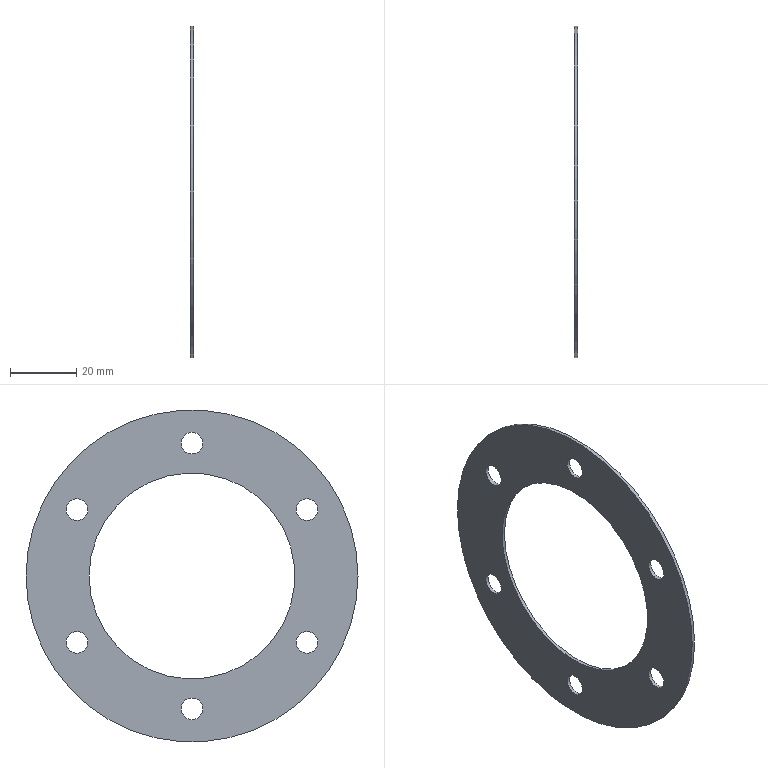Component | NX | DADIANPIAN | 1 solid | 10 faces | box 1 x 100 x 100 mm | volume 4636 mm3 | cylinder 8 | plane 2 | commonest cylinder face diameters 6.5 x6 100 x1 62 x1
STEP:
#1=CARTESIAN_POINT('',(0.,0.,0.));
#2=DIRECTION('',(0.,0.,1.));
#3=DIRECTION('',(1.,0.,0.));
#4=AXIS2_PLACEMENT_3D('',#1,#2,#3);
#5=CARTESIAN_POINT('',(111.,250.,-88.));
#6=VERTEX_POINT('',#5);
#7=CARTESIAN_POINT('',(111.,200.,-88.));
#8=DIRECTION('',(1.,0.,0.));
#9=DIRECTION('',(0.,1.,0.));
#10=AXIS2_PLACEMENT_3D('',#7,#8,#9);
#11=CIRCLE('',#10,50.);
#12=CARTESIAN_POINT('',(111.,200.,-88.));
#13=DIRECTION('',(-1.,0.,0.));
#14=DIRECTION('',(0.,0.,1.));
#15=AXIS2_PLACEMENT_3D('',#12,#13,#14);
#16=CYLINDRICAL_SURFACE('',#15,50.);
#17=CARTESIAN_POINT('',(7.854,0.));
#18=DIRECTION('',(-1.,0.));
#19=VECTOR('',#18,1.);
#20=LINE('',#17,#19);
#21=(GEOMETRIC_REPRESENTATION_CONTEXT(2)PARAMETRIC_REPRESENTATION_CONTEXT()REPRESENTATION_CONTEXT('',''));
#22=DEFINITIONAL_REPRESENTATION('',(#20),#21);
#23=PCURVE('',#16,#22);
#24=CARTESIAN_POINT('',(111.,200.,-88.));
#25=DIRECTION('',(1.,0.,0.));
#26=DIRECTION('',(0.,0.,-1.));
#27=AXIS2_PLACEMENT_3D('',#24,#25,#26);
#28=PLANE('',#27);
#29=CARTESIAN_POINT('',(0.,0.));
#30=DIRECTION('',(0.,1.));
#31=AXIS2_PLACEMENT_2D('',#29,#30);
#32=CIRCLE('',#31,50.);
#33=(GEOMETRIC_REPRESENTATION_CONTEXT(2)PARAMETRIC_REPRESENTATION_CONTEXT()REPRESENTATION_CONTEXT('',''));
#34=DEFINITIONAL_REPRESENTATION('',(#32),#33);
#35=PCURVE('',#28,#34);
#36=SURFACE_CURVE('',#11,(#23,#35),.PCURVE_S1.);
#37=EDGE_CURVE('',#6,#6,#36,.T.);
#38=ORIENTED_EDGE('',*,*,#37,.F.);
#39=CARTESIAN_POINT('',(110.,250.,-88.));
#40=VERTEX_POINT('',#39);
#41=CARTESIAN_POINT('',(111.,250.,-88.));
#42=CARTESIAN_POINT('',(110.,250.,-88.));
#43=B_SPLINE_CURVE_WITH_KNOTS('',1,(#41,#42),.UNSPECIFIED.,.F.,.F.,(2,2),(0.,1.),.PIECEWISE_BEZIER_KNOTS.);
#44=CARTESIAN_POINT('',(7.854,0.));
#45=DIRECTION('',(0.,1.));
#46=VECTOR('',#45,1.);
#47=LINE('',#44,#46);
#48=(GEOMETRIC_REPRESENTATION_CONTEXT(2)PARAMETRIC_REPRESENTATION_CONTEXT()REPRESENTATION_CONTEXT('',''));
#49=DEFINITIONAL_REPRESENTATION('',(#47),#48);
#50=PCURVE('',#16,#49);
#51=CARTESIAN_POINT('',(1.571,0.));
#52=DIRECTION('',(0.,1.));
#53=VECTOR('',#52,1.);
#54=LINE('',#51,#53);
#55=(GEOMETRIC_REPRESENTATION_CONTEXT(2)PARAMETRIC_REPRESENTATION_CONTEXT()REPRESENTATION_CONTEXT('',''));
#56=DEFINITIONAL_REPRESENTATION('',(#54),#55);
#57=PCURVE('',#16,#56);
#58=SEAM_CURVE('',#43,(#50,#57),.PCURVE_S1.);
#59=EDGE_CURVE('',#6,#40,#58,.T.);
#60=ORIENTED_EDGE('',*,*,#59,.T.);
#61=CARTESIAN_POINT('',(110.,200.,-88.));
#62=DIRECTION('',(1.,0.,0.));
#63=DIRECTION('',(0.,1.,0.));
#64=AXIS2_PLACEMENT_3D('',#61,#62,#63);
#65=CIRCLE('',#64,50.);
#66=CARTESIAN_POINT('',(7.854,1.));
#67=DIRECTION('',(-1.,0.));
#68=VECTOR('',#67,1.);
#69=LINE('',#66,#68);
#70=(GEOMETRIC_REPRESENTATION_CONTEXT(2)PARAMETRIC_REPRESENTATION_CONTEXT()REPRESENTATION_CONTEXT('',''));
#71=DEFINITIONAL_REPRESENTATION('',(#69),#70);
#72=PCURVE('',#16,#71);
#73=CARTESIAN_POINT('',(110.,200.,-88.));
#74=DIRECTION('',(1.,0.,0.));
#75=DIRECTION('',(0.,0.,-1.));
#76=AXIS2_PLACEMENT_3D('',#73,#74,#75);
#77=PLANE('',#76);
#78=CARTESIAN_POINT('',(0.,0.));
#79=DIRECTION('',(0.,1.));
#80=AXIS2_PLACEMENT_2D('',#78,#79);
#81=CIRCLE('',#80,50.);
#82=(GEOMETRIC_REPRESENTATION_CONTEXT(2)PARAMETRIC_REPRESENTATION_CONTEXT()REPRESENTATION_CONTEXT('',''));
#83=DEFINITIONAL_REPRESENTATION('',(#81),#82);
#84=PCURVE('',#77,#83);
#85=SURFACE_CURVE('',#65,(#72,#84),.PCURVE_S1.);
#86=EDGE_CURVE('',#40,#40,#85,.T.);
#87=ORIENTED_EDGE('',*,*,#86,.T.);
#88=ORIENTED_EDGE('',*,*,#59,.F.);
#89=EDGE_LOOP('',(#38,#60,#87,#88));
#90=FACE_BOUND('',#89,.T.);
#91=ADVANCED_FACE('',(#90),#16,.T.);
#92=CARTESIAN_POINT('',(111.,231.,-88.));
#93=VERTEX_POINT('',#92);
#94=CARTESIAN_POINT('',(111.,200.,-88.));
#95=DIRECTION('',(1.,0.,0.));
#96=DIRECTION('',(0.,1.,0.));
#97=AXIS2_PLACEMENT_3D('',#94,#95,#96);
#98=CIRCLE('',#97,31.);
#99=CARTESIAN_POINT('',(111.,200.,-88.));
#100=DIRECTION('',(-1.,0.,0.));
#101=DIRECTION('',(0.,0.,1.));
#102=AXIS2_PLACEMENT_3D('',#99,#100,#101);
#103=CYLINDRICAL_SURFACE('',#102,31.);
#104=CARTESIAN_POINT('',(7.854,0.));
#105=DIRECTION('',(-1.,0.));
#106=VECTOR('',#105,1.);
#107=LINE('',#104,#106);
#108=(GEOMETRIC_REPRESENTATION_CONTEXT(2)PARAMETRIC_REPRESENTATION_CONTEXT()REPRESENTATION_CONTEXT('',''));
#109=DEFINITIONAL_REPRESENTATION('',(#107),#108);
#110=PCURVE('',#103,#109);
#111=CARTESIAN_POINT('',(0.,0.));
#112=DIRECTION('',(0.,1.));
#113=AXIS2_PLACEMENT_2D('',#111,#112);
#114=CIRCLE('',#113,31.);
#115=(GEOMETRIC_REPRESENTATION_CONTEXT(2)PARAMETRIC_REPRESENTATION_CONTEXT()REPRESENTATION_CONTEXT('',''));
#116=DEFINITIONAL_REPRESENTATION('',(#114),#115);
#117=PCURVE('',#28,#116);
#118=SURFACE_CURVE('',#98,(#110,#117),.PCURVE_S1.);
#119=EDGE_CURVE('',#93,#93,#118,.T.);
#120=ORIENTED_EDGE('',*,*,#119,.F.);
#121=CARTESIAN_POINT('',(110.,231.,-88.));
#122=VERTEX_POINT('',#121);
#123=CARTESIAN_POINT('',(111.,231.,-88.));
#124=CARTESIAN_POINT('',(110.,231.,-88.));
#125=B_SPLINE_CURVE_WITH_KNOTS('',1,(#123,#124),.UNSPECIFIED.,.F.,.F.,(2,2),(0.,1.),.PIECEWISE_BEZIER_KNOTS.);
#126=CARTESIAN_POINT('',(7.854,0.));
#127=DIRECTION('',(0.,1.));
#128=VECTOR('',#127,1.);
#129=LINE('',#126,#128);
#130=(GEOMETRIC_REPRESENTATION_CONTEXT(2)PARAMETRIC_REPRESENTATION_CONTEXT()REPRESENTATION_CONTEXT('',''));
#131=DEFINITIONAL_REPRESENTATION('',(#129),#130);
#132=PCURVE('',#103,#131);
#133=CARTESIAN_POINT('',(1.571,0.));
#134=DIRECTION('',(0.,1.));
#135=VECTOR('',#134,1.);
#136=LINE('',#133,#135);
#137=(GEOMETRIC_REPRESENTATION_CONTEXT(2)PARAMETRIC_REPRESENTATION_CONTEXT()REPRESENTATION_CONTEXT('',''));
#138=DEFINITIONAL_REPRESENTATION('',(#136),#137);
#139=PCURVE('',#103,#138);
#140=SEAM_CURVE('',#125,(#132,#139),.PCURVE_S1.);
#141=EDGE_CURVE('',#93,#122,#140,.T.);
#142=ORIENTED_EDGE('',*,*,#141,.T.);
#143=CARTESIAN_POINT('',(110.,200.,-88.));
#144=DIRECTION('',(1.,0.,0.));
#145=DIRECTION('',(0.,1.,0.));
#146=AXIS2_PLACEMENT_3D('',#143,#144,#145);
#147=CIRCLE('',#146,31.);
#148=CARTESIAN_POINT('',(7.854,1.));
#149=DIRECTION('',(-1.,0.));
#150=VECTOR('',#149,1.);
#151=LINE('',#148,#150);
#152=(GEOMETRIC_REPRESENTATION_CONTEXT(2)PARAMETRIC_REPRESENTATION_CONTEXT()REPRESENTATION_CONTEXT('',''));
#153=DEFINITIONAL_REPRESENTATION('',(#151),#152);
#154=PCURVE('',#103,#153);
#155=CARTESIAN_POINT('',(0.,0.));
#156=DIRECTION('',(0.,1.));
#157=AXIS2_PLACEMENT_2D('',#155,#156);
#158=CIRCLE('',#157,31.);
#159=(GEOMETRIC_REPRESENTATION_CONTEXT(2)PARAMETRIC_REPRESENTATION_CONTEXT()REPRESENTATION_CONTEXT('',''));
#160=DEFINITIONAL_REPRESENTATION('',(#158),#159);
#161=PCURVE('',#77,#160);
#162=SURFACE_CURVE('',#147,(#154,#161),.PCURVE_S1.);
#163=EDGE_CURVE('',#122,#122,#162,.T.);
#164=ORIENTED_EDGE('',*,*,#163,.T.);
#165=ORIENTED_EDGE('',*,*,#141,.F.);
#166=EDGE_LOOP('',(#120,#142,#164,#165));
#167=FACE_BOUND('',#166,.F.);
#168=ADVANCED_FACE('',(#167),#103,.F.);
#169=CARTESIAN_POINT('',(111.,234.641,-64.75));
#170=VERTEX_POINT('',#169);
#171=CARTESIAN_POINT('',(111.,234.641,-68.));
#172=DIRECTION('',(-1.,0.,0.));
#173=DIRECTION('',(0.,0.,1.));
#174=AXIS2_PLACEMENT_3D('',#171,#172,#173);
#175=CIRCLE('',#174,3.25);
#176=CARTESIAN_POINT('',(-23.25,34.641));
#177=CARTESIAN_POINT('',(-23.25,40.27));
#178=CARTESIAN_POINT('',(-18.375,37.456));
#179=CARTESIAN_POINT('',(-13.5,34.641));
#180=CARTESIAN_POINT('',(-18.375,31.826));
#181=CARTESIAN_POINT('',(-23.25,29.012));
#182=CARTESIAN_POINT('',(-23.25,34.641));
#183=(BOUNDED_CURVE()B_SPLINE_CURVE(2,(#176,#177,#178,#179,#180,#181,#182),.UNSPECIFIED.,.T.,.F.)B_SPLINE_CURVE_WITH_KNOTS((1,2,2,2,2,1),(-2.094,0.,2.094,4.189,6.283,8.378),.UNSPECIFIED.)CURVE()GEOMETRIC_REPRESENTATION_ITEM()RATIONAL_B_SPLINE_CURVE((1.,0.5,1.,0.5,1.,0.5,1.))REPRESENTATION_ITEM(''));
#184=(GEOMETRIC_REPRESENTATION_CONTEXT(2)PARAMETRIC_REPRESENTATION_CONTEXT()REPRESENTATION_CONTEXT('',''));
#185=DEFINITIONAL_REPRESENTATION('',(#183),#184);
#186=PCURVE('',#28,#185);
#187=CARTESIAN_POINT('',(111.,234.641,-68.));
#188=DIRECTION('',(-1.,0.,0.));
#189=DIRECTION('',(0.,0.,1.));
#190=AXIS2_PLACEMENT_3D('',#187,#188,#189);
#191=CYLINDRICAL_SURFACE('',#190,3.25);
#192=CARTESIAN_POINT('',(0.,0.));
#193=DIRECTION('',(1.,0.));
#194=VECTOR('',#193,1.);
#195=LINE('',#192,#194);
#196=(GEOMETRIC_REPRESENTATION_CONTEXT(2)PARAMETRIC_REPRESENTATION_CONTEXT()REPRESENTATION_CONTEXT('',''));
#197=DEFINITIONAL_REPRESENTATION('',(#195),#196);
#198=PCURVE('',#191,#197);
#199=SURFACE_CURVE('',#175,(#186,#198),.PCURVE_S1.);
#200=EDGE_CURVE('',#170,#170,#199,.T.);
#201=ORIENTED_EDGE('',*,*,#200,.T.);
#202=EDGE_LOOP('',(#201));
#203=FACE_BOUND('',#202,.T.);
#204=CARTESIAN_POINT('',(111.,234.641,-104.75));
#205=VERTEX_POINT('',#204);
#206=CARTESIAN_POINT('',(111.,234.641,-108.));
#207=DIRECTION('',(-1.,0.,0.));
#208=DIRECTION('',(0.,0.,1.));
#209=AXIS2_PLACEMENT_3D('',#206,#207,#208);
#210=CIRCLE('',#209,3.25);
#211=CARTESIAN_POINT('',(16.75,34.641));
#212=CARTESIAN_POINT('',(16.75,40.27));
#213=CARTESIAN_POINT('',(21.625,37.456));
#214=CARTESIAN_POINT('',(26.5,34.641));
#215=CARTESIAN_POINT('',(21.625,31.826));
#216=CARTESIAN_POINT('',(16.75,29.012));
#217=CARTESIAN_POINT('',(16.75,34.641));
#218=(BOUNDED_CURVE()B_SPLINE_CURVE(2,(#211,#212,#213,#214,#215,#216,#217),.UNSPECIFIED.,.T.,.F.)B_SPLINE_CURVE_WITH_KNOTS((1,2,2,2,2,1),(-2.094,0.,2.094,4.189,6.283,8.378),.UNSPECIFIED.)CURVE()GEOMETRIC_REPRESENTATION_ITEM()RATIONAL_B_SPLINE_CURVE((1.,0.5,1.,0.5,1.,0.5,1.))REPRESENTATION_ITEM(''));
#219=(GEOMETRIC_REPRESENTATION_CONTEXT(2)PARAMETRIC_REPRESENTATION_CONTEXT()REPRESENTATION_CONTEXT('',''));
#220=DEFINITIONAL_REPRESENTATION('',(#218),#219);
#221=PCURVE('',#28,#220);
#222=CARTESIAN_POINT('',(111.,234.641,-108.));
#223=DIRECTION('',(-1.,0.,0.));
#224=DIRECTION('',(0.,0.,1.));
#225=AXIS2_PLACEMENT_3D('',#222,#223,#224);
#226=CYLINDRICAL_SURFACE('',#225,3.25);
#227=CARTESIAN_POINT('',(0.,0.));
#228=DIRECTION('',(1.,0.));
#229=VECTOR('',#228,1.);
#230=LINE('',#227,#229);
#231=(GEOMETRIC_REPRESENTATION_CONTEXT(2)PARAMETRIC_REPRESENTATION_CONTEXT()REPRESENTATION_CONTEXT('',''));
#232=DEFINITIONAL_REPRESENTATION('',(#230),#231);
#233=PCURVE('',#226,#232);
#234=SURFACE_CURVE('',#210,(#221,#233),.PCURVE_S1.);
#235=EDGE_CURVE('',#205,#205,#234,.T.);
#236=ORIENTED_EDGE('',*,*,#235,.T.);
#237=EDGE_LOOP('',(#236));
#238=FACE_BOUND('',#237,.T.);
#239=CARTESIAN_POINT('',(111.,200.,-44.75));
#240=VERTEX_POINT('',#239);
#241=CARTESIAN_POINT('',(111.,200.,-48.));
#242=DIRECTION('',(-1.,0.,0.));
#243=DIRECTION('',(0.,0.,1.));
#244=AXIS2_PLACEMENT_3D('',#241,#242,#243);
#245=CIRCLE('',#244,3.25);
#246=CARTESIAN_POINT('',(-43.25,0.));
#247=CARTESIAN_POINT('',(-43.25,5.629));
#248=CARTESIAN_POINT('',(-38.375,2.815));
#249=CARTESIAN_POINT('',(-33.5,0.));
#250=CARTESIAN_POINT('',(-38.375,-2.815));
#251=CARTESIAN_POINT('',(-43.25,-5.629));
#252=CARTESIAN_POINT('',(-43.25,0.));
#253=(BOUNDED_CURVE()B_SPLINE_CURVE(2,(#246,#247,#248,#249,#250,#251,#252),.UNSPECIFIED.,.T.,.F.)B_SPLINE_CURVE_WITH_KNOTS((1,2,2,2,2,1),(-2.094,0.,2.094,4.189,6.283,8.378),.UNSPECIFIED.)CURVE()GEOMETRIC_REPRESENTATION_ITEM()RATIONAL_B_SPLINE_CURVE((1.,0.5,1.,0.5,1.,0.5,1.))REPRESENTATION_ITEM(''));
#254=(GEOMETRIC_REPRESENTATION_CONTEXT(2)PARAMETRIC_REPRESENTATION_CONTEXT()REPRESENTATION_CONTEXT('',''));
#255=DEFINITIONAL_REPRESENTATION('',(#253),#254);
#256=PCURVE('',#28,#255);
#257=CARTESIAN_POINT('',(111.,200.,-48.));
#258=DIRECTION('',(-1.,0.,0.));
#259=DIRECTION('',(0.,0.,1.));
#260=AXIS2_PLACEMENT_3D('',#257,#258,#259);
#261=CYLINDRICAL_SURFACE('',#260,3.25);
#262=CARTESIAN_POINT('',(0.,0.));
#263=DIRECTION('',(1.,0.));
#264=VECTOR('',#263,1.);
#265=LINE('',#262,#264);
#266=(GEOMETRIC_REPRESENTATION_CONTEXT(2)PARAMETRIC_REPRESENTATION_CONTEXT()REPRESENTATION_CONTEXT('',''));
#267=DEFINITIONAL_REPRESENTATION('',(#265),#266);
#268=PCURVE('',#261,#267);
#269=SURFACE_CURVE('',#245,(#256,#268),.PCURVE_S1.);
#270=EDGE_CURVE('',#240,#240,#269,.T.);
#271=ORIENTED_EDGE('',*,*,#270,.T.);
#272=EDGE_LOOP('',(#271));
#273=FACE_BOUND('',#272,.T.);
#274=CARTESIAN_POINT('',(111.,200.,-124.75));
#275=VERTEX_POINT('',#274);
#276=CARTESIAN_POINT('',(111.,200.,-128.));
#277=DIRECTION('',(-1.,0.,0.));
#278=DIRECTION('',(0.,0.,1.));
#279=AXIS2_PLACEMENT_3D('',#276,#277,#278);
#280=CIRCLE('',#279,3.25);
#281=CARTESIAN_POINT('',(36.75,0.));
#282=CARTESIAN_POINT('',(36.75,5.629));
#283=CARTESIAN_POINT('',(41.625,2.815));
#284=CARTESIAN_POINT('',(46.5,0.));
#285=CARTESIAN_POINT('',(41.625,-2.815));
#286=CARTESIAN_POINT('',(36.75,-5.629));
#287=CARTESIAN_POINT('',(36.75,0.));
#288=(BOUNDED_CURVE()B_SPLINE_CURVE(2,(#281,#282,#283,#284,#285,#286,#287),.UNSPECIFIED.,.T.,.F.)B_SPLINE_CURVE_WITH_KNOTS((1,2,2,2,2,1),(-2.094,0.,2.094,4.189,6.283,8.378),.UNSPECIFIED.)CURVE()GEOMETRIC_REPRESENTATION_ITEM()RATIONAL_B_SPLINE_CURVE((1.,0.5,1.,0.5,1.,0.5,1.))REPRESENTATION_ITEM(''));
#289=(GEOMETRIC_REPRESENTATION_CONTEXT(2)PARAMETRIC_REPRESENTATION_CONTEXT()REPRESENTATION_CONTEXT('',''));
#290=DEFINITIONAL_REPRESENTATION('',(#288),#289);
#291=PCURVE('',#28,#290);
#292=CARTESIAN_POINT('',(111.,200.,-128.));
#293=DIRECTION('',(-1.,0.,0.));
#294=DIRECTION('',(0.,0.,1.));
#295=AXIS2_PLACEMENT_3D('',#292,#293,#294);
#296=CYLINDRICAL_SURFACE('',#295,3.25);
#297=CARTESIAN_POINT('',(0.,0.));
#298=DIRECTION('',(1.,0.));
#299=VECTOR('',#298,1.);
#300=LINE('',#297,#299);
#301=(GEOMETRIC_REPRESENTATION_CONTEXT(2)PARAMETRIC_REPRESENTATION_CONTEXT()REPRESENTATION_CONTEXT('',''));
#302=DEFINITIONAL_REPRESENTATION('',(#300),#301);
#303=PCURVE('',#296,#302);
#304=SURFACE_CURVE('',#280,(#291,#303),.PCURVE_S1.);
#305=EDGE_CURVE('',#275,#275,#304,.T.);
#306=ORIENTED_EDGE('',*,*,#305,.T.);
#307=EDGE_LOOP('',(#306));
#308=FACE_BOUND('',#307,.T.);
#309=CARTESIAN_POINT('',(111.,165.359,-64.75));
#310=VERTEX_POINT('',#309);
#311=CARTESIAN_POINT('',(111.,165.359,-68.));
#312=DIRECTION('',(-1.,0.,0.));
#313=DIRECTION('',(0.,0.,1.));
#314=AXIS2_PLACEMENT_3D('',#311,#312,#313);
#315=CIRCLE('',#314,3.25);
#316=CARTESIAN_POINT('',(-23.25,-34.641));
#317=CARTESIAN_POINT('',(-23.25,-29.012));
#318=CARTESIAN_POINT('',(-18.375,-31.826));
#319=CARTESIAN_POINT('',(-13.5,-34.641));
#320=CARTESIAN_POINT('',(-18.375,-37.456));
#321=CARTESIAN_POINT('',(-23.25,-40.27));
#322=CARTESIAN_POINT('',(-23.25,-34.641));
#323=(BOUNDED_CURVE()B_SPLINE_CURVE(2,(#316,#317,#318,#319,#320,#321,#322),.UNSPECIFIED.,.T.,.F.)B_SPLINE_CURVE_WITH_KNOTS((1,2,2,2,2,1),(-2.094,0.,2.094,4.189,6.283,8.378),.UNSPECIFIED.)CURVE()GEOMETRIC_REPRESENTATION_ITEM()RATIONAL_B_SPLINE_CURVE((1.,0.5,1.,0.5,1.,0.5,1.))REPRESENTATION_ITEM(''));
#324=(GEOMETRIC_REPRESENTATION_CONTEXT(2)PARAMETRIC_REPRESENTATION_CONTEXT()REPRESENTATION_CONTEXT('',''));
#325=DEFINITIONAL_REPRESENTATION('',(#323),#324);
#326=PCURVE('',#28,#325);
#327=CARTESIAN_POINT('',(111.,165.359,-68.));
#328=DIRECTION('',(-1.,0.,0.));
#329=DIRECTION('',(0.,0.,1.));
#330=AXIS2_PLACEMENT_3D('',#327,#328,#329);
#331=CYLINDRICAL_SURFACE('',#330,3.25);
#332=CARTESIAN_POINT('',(0.,0.));
#333=DIRECTION('',(1.,0.));
#334=VECTOR('',#333,1.);
#335=LINE('',#332,#334);
#336=(GEOMETRIC_REPRESENTATION_CONTEXT(2)PARAMETRIC_REPRESENTATION_CONTEXT()REPRESENTATION_CONTEXT('',''));
#337=DEFINITIONAL_REPRESENTATION('',(#335),#336);
#338=PCURVE('',#331,#337);
#339=SURFACE_CURVE('',#315,(#326,#338),.PCURVE_S1.);
#340=EDGE_CURVE('',#310,#310,#339,.T.);
#341=ORIENTED_EDGE('',*,*,#340,.T.);
#342=EDGE_LOOP('',(#341));
#343=FACE_BOUND('',#342,.T.);
#344=CARTESIAN_POINT('',(111.,165.359,-104.75));
#345=VERTEX_POINT('',#344);
#346=CARTESIAN_POINT('',(111.,165.359,-108.));
#347=DIRECTION('',(-1.,0.,0.));
#348=DIRECTION('',(0.,0.,1.));
#349=AXIS2_PLACEMENT_3D('',#346,#347,#348);
#350=CIRCLE('',#349,3.25);
#351=CARTESIAN_POINT('',(16.75,-34.641));
#352=CARTESIAN_POINT('',(16.75,-29.012));
#353=CARTESIAN_POINT('',(21.625,-31.826));
#354=CARTESIAN_POINT('',(26.5,-34.641));
#355=CARTESIAN_POINT('',(21.625,-37.456));
#356=CARTESIAN_POINT('',(16.75,-40.27));
#357=CARTESIAN_POINT('',(16.75,-34.641));
#358=(BOUNDED_CURVE()B_SPLINE_CURVE(2,(#351,#352,#353,#354,#355,#356,#357),.UNSPECIFIED.,.T.,.F.)B_SPLINE_CURVE_WITH_KNOTS((1,2,2,2,2,1),(-2.094,0.,2.094,4.189,6.283,8.378),.UNSPECIFIED.)CURVE()GEOMETRIC_REPRESENTATION_ITEM()RATIONAL_B_SPLINE_CURVE((1.,0.5,1.,0.5,1.,0.5,1.))REPRESENTATION_ITEM(''));
#359=(GEOMETRIC_REPRESENTATION_CONTEXT(2)PARAMETRIC_REPRESENTATION_CONTEXT()REPRESENTATION_CONTEXT('',''));
#360=DEFINITIONAL_REPRESENTATION('',(#358),#359);
#361=PCURVE('',#28,#360);
#362=CARTESIAN_POINT('',(111.,165.359,-108.));
#363=DIRECTION('',(-1.,0.,0.));
#364=DIRECTION('',(0.,0.,1.));
#365=AXIS2_PLACEMENT_3D('',#362,#363,#364);
#366=CYLINDRICAL_SURFACE('',#365,3.25);
#367=CARTESIAN_POINT('',(0.,0.));
#368=DIRECTION('',(1.,0.));
#369=VECTOR('',#368,1.);
#370=LINE('',#367,#369);
#371=(GEOMETRIC_REPRESENTATION_CONTEXT(2)PARAMETRIC_REPRESENTATION_CONTEXT()REPRESENTATION_CONTEXT('',''));
#372=DEFINITIONAL_REPRESENTATION('',(#370),#371);
#373=PCURVE('',#366,#372);
#374=SURFACE_CURVE('',#350,(#361,#373),.PCURVE_S1.);
#375=EDGE_CURVE('',#345,#345,#374,.T.);
#376=ORIENTED_EDGE('',*,*,#375,.T.);
#377=EDGE_LOOP('',(#376));
#378=FACE_BOUND('',#377,.T.);
#379=ORIENTED_EDGE('',*,*,#37,.T.);
#380=EDGE_LOOP('',(#379));
#381=FACE_BOUND('',#380,.T.);
#382=ORIENTED_EDGE('',*,*,#119,.F.);
#383=EDGE_LOOP('',(#382));
#384=FACE_BOUND('',#383,.T.);
#385=ADVANCED_FACE('',(#203,#238,#273,#308,#343,#378,#381,#384),#28,.T.);
#386=CARTESIAN_POINT('',(110.,234.641,-71.25));
#387=VERTEX_POINT('',#386);
#388=CARTESIAN_POINT('',(110.,234.641,-64.75));
#389=VERTEX_POINT('',#388);
#390=CARTESIAN_POINT('',(110.,234.641,-68.));
#391=DIRECTION('',(1.,0.,0.));
#392=DIRECTION('',(0.,0.,-1.));
#393=AXIS2_PLACEMENT_3D('',#390,#391,#392);
#394=CIRCLE('',#393,3.25);
#395=CARTESIAN_POINT('',(-20.,34.641));
#396=DIRECTION('',(1.,0.));
#397=AXIS2_PLACEMENT_2D('',#395,#396);
#398=CIRCLE('',#397,3.25);
#399=(GEOMETRIC_REPRESENTATION_CONTEXT(2)PARAMETRIC_REPRESENTATION_CONTEXT()REPRESENTATION_CONTEXT('',''));
#400=DEFINITIONAL_REPRESENTATION('',(#398),#399);
#401=PCURVE('',#77,#400);
#402=CARTESIAN_POINT('',(3.142,1.));
#403=DIRECTION('',(-1.,0.));
#404=VECTOR('',#403,1.);
#405=LINE('',#402,#404);
#406=(GEOMETRIC_REPRESENTATION_CONTEXT(2)PARAMETRIC_REPRESENTATION_CONTEXT()REPRESENTATION_CONTEXT('',''));
#407=DEFINITIONAL_REPRESENTATION('',(#405),#406);
#408=PCURVE('',#191,#407);
#409=SURFACE_CURVE('',#394,(#401,#408),.PCURVE_S1.);
#410=EDGE_CURVE('',#387,#389,#409,.T.);
#411=ORIENTED_EDGE('',*,*,#410,.T.);
#412=CARTESIAN_POINT('',(110.,234.641,-68.));
#413=DIRECTION('',(1.,0.,0.));
#414=DIRECTION('',(0.,0.,-1.));
#415=AXIS2_PLACEMENT_3D('',#412,#413,#414);
#416=CIRCLE('',#415,3.25);
#417=CARTESIAN_POINT('',(-20.,34.641));
#418=DIRECTION('',(1.,0.));
#419=AXIS2_PLACEMENT_2D('',#417,#418);
#420=CIRCLE('',#419,3.25);
#421=(GEOMETRIC_REPRESENTATION_CONTEXT(2)PARAMETRIC_REPRESENTATION_CONTEXT()REPRESENTATION_CONTEXT('',''));
#422=DEFINITIONAL_REPRESENTATION('',(#420),#421);
#423=PCURVE('',#77,#422);
#424=CARTESIAN_POINT('',(9.425,1.));
#425=DIRECTION('',(-1.,0.));
#426=VECTOR('',#425,1.);
#427=LINE('',#424,#426);
#428=(GEOMETRIC_REPRESENTATION_CONTEXT(2)PARAMETRIC_REPRESENTATION_CONTEXT()REPRESENTATION_CONTEXT('',''));
#429=DEFINITIONAL_REPRESENTATION('',(#427),#428);
#430=PCURVE('',#191,#429);
#431=SURFACE_CURVE('',#416,(#423,#430),.PCURVE_S1.);
#432=EDGE_CURVE('',#389,#387,#431,.T.);
#433=ORIENTED_EDGE('',*,*,#432,.T.);
#434=EDGE_LOOP('',(#411,#433));
#435=FACE_BOUND('',#434,.T.);
#436=CARTESIAN_POINT('',(110.,234.641,-111.25));
#437=VERTEX_POINT('',#436);
#438=CARTESIAN_POINT('',(110.,234.641,-104.75));
#439=VERTEX_POINT('',#438);
#440=CARTESIAN_POINT('',(110.,234.641,-108.));
#441=DIRECTION('',(1.,0.,0.));
#442=DIRECTION('',(0.,0.,-1.));
#443=AXIS2_PLACEMENT_3D('',#440,#441,#442);
#444=CIRCLE('',#443,3.25);
#445=CARTESIAN_POINT('',(20.,34.641));
#446=DIRECTION('',(1.,0.));
#447=AXIS2_PLACEMENT_2D('',#445,#446);
#448=CIRCLE('',#447,3.25);
#449=(GEOMETRIC_REPRESENTATION_CONTEXT(2)PARAMETRIC_REPRESENTATION_CONTEXT()REPRESENTATION_CONTEXT('',''));
#450=DEFINITIONAL_REPRESENTATION('',(#448),#449);
#451=PCURVE('',#77,#450);
#452=CARTESIAN_POINT('',(3.142,1.));
#453=DIRECTION('',(-1.,0.));
#454=VECTOR('',#453,1.);
#455=LINE('',#452,#454);
#456=(GEOMETRIC_REPRESENTATION_CONTEXT(2)PARAMETRIC_REPRESENTATION_CONTEXT()REPRESENTATION_CONTEXT('',''));
#457=DEFINITIONAL_REPRESENTATION('',(#455),#456);
#458=PCURVE('',#226,#457);
#459=SURFACE_CURVE('',#444,(#451,#458),.PCURVE_S1.);
#460=EDGE_CURVE('',#437,#439,#459,.T.);
#461=ORIENTED_EDGE('',*,*,#460,.T.);
#462=CARTESIAN_POINT('',(110.,234.641,-108.));
#463=DIRECTION('',(1.,0.,0.));
#464=DIRECTION('',(0.,0.,-1.));
#465=AXIS2_PLACEMENT_3D('',#462,#463,#464);
#466=CIRCLE('',#465,3.25);
#467=CARTESIAN_POINT('',(20.,34.641));
#468=DIRECTION('',(1.,0.));
#469=AXIS2_PLACEMENT_2D('',#467,#468);
#470=CIRCLE('',#469,3.25);
#471=(GEOMETRIC_REPRESENTATION_CONTEXT(2)PARAMETRIC_REPRESENTATION_CONTEXT()REPRESENTATION_CONTEXT('',''));
#472=DEFINITIONAL_REPRESENTATION('',(#470),#471);
#473=PCURVE('',#77,#472);
#474=CARTESIAN_POINT('',(9.425,1.));
#475=DIRECTION('',(-1.,0.));
#476=VECTOR('',#475,1.);
#477=LINE('',#474,#476);
#478=(GEOMETRIC_REPRESENTATION_CONTEXT(2)PARAMETRIC_REPRESENTATION_CONTEXT()REPRESENTATION_CONTEXT('',''));
#479=DEFINITIONAL_REPRESENTATION('',(#477),#478);
#480=PCURVE('',#226,#479);
#481=SURFACE_CURVE('',#466,(#473,#480),.PCURVE_S1.);
#482=EDGE_CURVE('',#439,#437,#481,.T.);
#483=ORIENTED_EDGE('',*,*,#482,.T.);
#484=EDGE_LOOP('',(#461,#483));
#485=FACE_BOUND('',#484,.T.);
#486=CARTESIAN_POINT('',(110.,200.,-51.25));
#487=VERTEX_POINT('',#486);
#488=CARTESIAN_POINT('',(110.,200.,-44.75));
#489=VERTEX_POINT('',#488);
#490=CARTESIAN_POINT('',(110.,200.,-48.));
#491=DIRECTION('',(1.,0.,0.));
#492=DIRECTION('',(0.,0.,-1.));
#493=AXIS2_PLACEMENT_3D('',#490,#491,#492);
#494=CIRCLE('',#493,3.25);
#495=CARTESIAN_POINT('',(-40.,0.));
#496=DIRECTION('',(1.,0.));
#497=AXIS2_PLACEMENT_2D('',#495,#496);
#498=CIRCLE('',#497,3.25);
#499=(GEOMETRIC_REPRESENTATION_CONTEXT(2)PARAMETRIC_REPRESENTATION_CONTEXT()REPRESENTATION_CONTEXT('',''));
#500=DEFINITIONAL_REPRESENTATION('',(#498),#499);
#501=PCURVE('',#77,#500);
#502=CARTESIAN_POINT('',(3.142,1.));
#503=DIRECTION('',(-1.,0.));
#504=VECTOR('',#503,1.);
#505=LINE('',#502,#504);
#506=(GEOMETRIC_REPRESENTATION_CONTEXT(2)PARAMETRIC_REPRESENTATION_CONTEXT()REPRESENTATION_CONTEXT('',''));
#507=DEFINITIONAL_REPRESENTATION('',(#505),#506);
#508=PCURVE('',#261,#507);
#509=SURFACE_CURVE('',#494,(#501,#508),.PCURVE_S1.);
#510=EDGE_CURVE('',#487,#489,#509,.T.);
#511=ORIENTED_EDGE('',*,*,#510,.T.);
#512=CARTESIAN_POINT('',(110.,200.,-48.));
#513=DIRECTION('',(1.,0.,0.));
#514=DIRECTION('',(0.,0.,-1.));
#515=AXIS2_PLACEMENT_3D('',#512,#513,#514);
#516=CIRCLE('',#515,3.25);
#517=CARTESIAN_POINT('',(-40.,0.));
#518=DIRECTION('',(1.,0.));
#519=AXIS2_PLACEMENT_2D('',#517,#518);
#520=CIRCLE('',#519,3.25);
#521=(GEOMETRIC_REPRESENTATION_CONTEXT(2)PARAMETRIC_REPRESENTATION_CONTEXT()REPRESENTATION_CONTEXT('',''));
#522=DEFINITIONAL_REPRESENTATION('',(#520),#521);
#523=PCURVE('',#77,#522);
#524=CARTESIAN_POINT('',(9.425,1.));
#525=DIRECTION('',(-1.,0.));
#526=VECTOR('',#525,1.);
#527=LINE('',#524,#526);
#528=(GEOMETRIC_REPRESENTATION_CONTEXT(2)PARAMETRIC_REPRESENTATION_CONTEXT()REPRESENTATION_CONTEXT('',''));
#529=DEFINITIONAL_REPRESENTATION('',(#527),#528);
#530=PCURVE('',#261,#529);
#531=SURFACE_CURVE('',#516,(#523,#530),.PCURVE_S1.);
#532=EDGE_CURVE('',#489,#487,#531,.T.);
#533=ORIENTED_EDGE('',*,*,#532,.T.);
#534=EDGE_LOOP('',(#511,#533));
#535=FACE_BOUND('',#534,.T.);
#536=CARTESIAN_POINT('',(110.,200.,-131.25));
#537=VERTEX_POINT('',#536);
#538=CARTESIAN_POINT('',(110.,200.,-124.75));
#539=VERTEX_POINT('',#538);
#540=CARTESIAN_POINT('',(110.,200.,-128.));
#541=DIRECTION('',(1.,0.,0.));
#542=DIRECTION('',(0.,0.,-1.));
#543=AXIS2_PLACEMENT_3D('',#540,#541,#542);
#544=CIRCLE('',#543,3.25);
#545=CARTESIAN_POINT('',(40.,0.));
#546=DIRECTION('',(1.,0.));
#547=AXIS2_PLACEMENT_2D('',#545,#546);
#548=CIRCLE('',#547,3.25);
#549=(GEOMETRIC_REPRESENTATION_CONTEXT(2)PARAMETRIC_REPRESENTATION_CONTEXT()REPRESENTATION_CONTEXT('',''));
#550=DEFINITIONAL_REPRESENTATION('',(#548),#549);
#551=PCURVE('',#77,#550);
#552=CARTESIAN_POINT('',(3.142,1.));
#553=DIRECTION('',(-1.,0.));
#554=VECTOR('',#553,1.);
#555=LINE('',#552,#554);
#556=(GEOMETRIC_REPRESENTATION_CONTEXT(2)PARAMETRIC_REPRESENTATION_CONTEXT()REPRESENTATION_CONTEXT('',''));
#557=DEFINITIONAL_REPRESENTATION('',(#555),#556);
#558=PCURVE('',#296,#557);
#559=SURFACE_CURVE('',#544,(#551,#558),.PCURVE_S1.);
#560=EDGE_CURVE('',#537,#539,#559,.T.);
#561=ORIENTED_EDGE('',*,*,#560,.T.);
#562=CARTESIAN_POINT('',(110.,200.,-128.));
#563=DIRECTION('',(1.,0.,0.));
#564=DIRECTION('',(0.,0.,-1.));
#565=AXIS2_PLACEMENT_3D('',#562,#563,#564);
#566=CIRCLE('',#565,3.25);
#567=CARTESIAN_POINT('',(40.,0.));
#568=DIRECTION('',(1.,0.));
#569=AXIS2_PLACEMENT_2D('',#567,#568);
#570=CIRCLE('',#569,3.25);
#571=(GEOMETRIC_REPRESENTATION_CONTEXT(2)PARAMETRIC_REPRESENTATION_CONTEXT()REPRESENTATION_CONTEXT('',''));
#572=DEFINITIONAL_REPRESENTATION('',(#570),#571);
#573=PCURVE('',#77,#572);
#574=CARTESIAN_POINT('',(9.425,1.));
#575=DIRECTION('',(-1.,0.));
#576=VECTOR('',#575,1.);
#577=LINE('',#574,#576);
#578=(GEOMETRIC_REPRESENTATION_CONTEXT(2)PARAMETRIC_REPRESENTATION_CONTEXT()REPRESENTATION_CONTEXT('',''));
#579=DEFINITIONAL_REPRESENTATION('',(#577),#578);
#580=PCURVE('',#296,#579);
#581=SURFACE_CURVE('',#566,(#573,#580),.PCURVE_S1.);
#582=EDGE_CURVE('',#539,#537,#581,.T.);
#583=ORIENTED_EDGE('',*,*,#582,.T.);
#584=EDGE_LOOP('',(#561,#583));
#585=FACE_BOUND('',#584,.T.);
#586=CARTESIAN_POINT('',(110.,165.359,-71.25));
#587=VERTEX_POINT('',#586);
#588=CARTESIAN_POINT('',(110.,165.359,-64.75));
#589=VERTEX_POINT('',#588);
#590=CARTESIAN_POINT('',(110.,165.359,-68.));
#591=DIRECTION('',(1.,0.,0.));
#592=DIRECTION('',(0.,0.,-1.));
#593=AXIS2_PLACEMENT_3D('',#590,#591,#592);
#594=CIRCLE('',#593,3.25);
#595=CARTESIAN_POINT('',(-20.,-34.641));
#596=DIRECTION('',(1.,0.));
#597=AXIS2_PLACEMENT_2D('',#595,#596);
#598=CIRCLE('',#597,3.25);
#599=(GEOMETRIC_REPRESENTATION_CONTEXT(2)PARAMETRIC_REPRESENTATION_CONTEXT()REPRESENTATION_CONTEXT('',''));
#600=DEFINITIONAL_REPRESENTATION('',(#598),#599);
#601=PCURVE('',#77,#600);
#602=CARTESIAN_POINT('',(3.142,1.));
#603=DIRECTION('',(-1.,0.));
#604=VECTOR('',#603,1.);
#605=LINE('',#602,#604);
#606=(GEOMETRIC_REPRESENTATION_CONTEXT(2)PARAMETRIC_REPRESENTATION_CONTEXT()REPRESENTATION_CONTEXT('',''));
#607=DEFINITIONAL_REPRESENTATION('',(#605),#606);
#608=PCURVE('',#331,#607);
#609=SURFACE_CURVE('',#594,(#601,#608),.PCURVE_S1.);
#610=EDGE_CURVE('',#587,#589,#609,.T.);
#611=ORIENTED_EDGE('',*,*,#610,.T.);
#612=CARTESIAN_POINT('',(110.,165.359,-68.));
#613=DIRECTION('',(1.,0.,0.));
#614=DIRECTION('',(0.,0.,-1.));
#615=AXIS2_PLACEMENT_3D('',#612,#613,#614);
#616=CIRCLE('',#615,3.25);
#617=CARTESIAN_POINT('',(-20.,-34.641));
#618=DIRECTION('',(1.,0.));
#619=AXIS2_PLACEMENT_2D('',#617,#618);
#620=CIRCLE('',#619,3.25);
#621=(GEOMETRIC_REPRESENTATION_CONTEXT(2)PARAMETRIC_REPRESENTATION_CONTEXT()REPRESENTATION_CONTEXT('',''));
#622=DEFINITIONAL_REPRESENTATION('',(#620),#621);
#623=PCURVE('',#77,#622);
#624=CARTESIAN_POINT('',(9.425,1.));
#625=DIRECTION('',(-1.,0.));
#626=VECTOR('',#625,1.);
#627=LINE('',#624,#626);
#628=(GEOMETRIC_REPRESENTATION_CONTEXT(2)PARAMETRIC_REPRESENTATION_CONTEXT()REPRESENTATION_CONTEXT('',''));
#629=DEFINITIONAL_REPRESENTATION('',(#627),#628);
#630=PCURVE('',#331,#629);
#631=SURFACE_CURVE('',#616,(#623,#630),.PCURVE_S1.);
#632=EDGE_CURVE('',#589,#587,#631,.T.);
#633=ORIENTED_EDGE('',*,*,#632,.T.);
#634=EDGE_LOOP('',(#611,#633));
#635=FACE_BOUND('',#634,.T.);
#636=CARTESIAN_POINT('',(110.,165.359,-111.25));
#637=VERTEX_POINT('',#636);
#638=CARTESIAN_POINT('',(110.,165.359,-104.75));
#639=VERTEX_POINT('',#638);
#640=CARTESIAN_POINT('',(110.,165.359,-108.));
#641=DIRECTION('',(1.,0.,0.));
#642=DIRECTION('',(0.,0.,-1.));
#643=AXIS2_PLACEMENT_3D('',#640,#641,#642);
#644=CIRCLE('',#643,3.25);
#645=CARTESIAN_POINT('',(20.,-34.641));
#646=DIRECTION('',(1.,0.));
#647=AXIS2_PLACEMENT_2D('',#645,#646);
#648=CIRCLE('',#647,3.25);
#649=(GEOMETRIC_REPRESENTATION_CONTEXT(2)PARAMETRIC_REPRESENTATION_CONTEXT()REPRESENTATION_CONTEXT('',''));
#650=DEFINITIONAL_REPRESENTATION('',(#648),#649);
#651=PCURVE('',#77,#650);
#652=CARTESIAN_POINT('',(3.142,1.));
#653=DIRECTION('',(-1.,0.));
#654=VECTOR('',#653,1.);
#655=LINE('',#652,#654);
#656=(GEOMETRIC_REPRESENTATION_CONTEXT(2)PARAMETRIC_REPRESENTATION_CONTEXT()REPRESENTATION_CONTEXT('',''));
#657=DEFINITIONAL_REPRESENTATION('',(#655),#656);
#658=PCURVE('',#366,#657);
#659=SURFACE_CURVE('',#644,(#651,#658),.PCURVE_S1.);
#660=EDGE_CURVE('',#637,#639,#659,.T.);
#661=ORIENTED_EDGE('',*,*,#660,.T.);
#662=CARTESIAN_POINT('',(110.,165.359,-108.));
#663=DIRECTION('',(1.,0.,0.));
#664=DIRECTION('',(0.,0.,-1.));
#665=AXIS2_PLACEMENT_3D('',#662,#663,#664);
#666=CIRCLE('',#665,3.25);
#667=CARTESIAN_POINT('',(20.,-34.641));
#668=DIRECTION('',(1.,0.));
#669=AXIS2_PLACEMENT_2D('',#667,#668);
#670=CIRCLE('',#669,3.25);
#671=(GEOMETRIC_REPRESENTATION_CONTEXT(2)PARAMETRIC_REPRESENTATION_CONTEXT()REPRESENTATION_CONTEXT('',''));
#672=DEFINITIONAL_REPRESENTATION('',(#670),#671);
#673=PCURVE('',#77,#672);
#674=CARTESIAN_POINT('',(9.425,1.));
#675=DIRECTION('',(-1.,0.));
#676=VECTOR('',#675,1.);
#677=LINE('',#674,#676);
#678=(GEOMETRIC_REPRESENTATION_CONTEXT(2)PARAMETRIC_REPRESENTATION_CONTEXT()REPRESENTATION_CONTEXT('',''));
#679=DEFINITIONAL_REPRESENTATION('',(#677),#678);
#680=PCURVE('',#366,#679);
#681=SURFACE_CURVE('',#666,(#673,#680),.PCURVE_S1.);
#682=EDGE_CURVE('',#639,#637,#681,.T.);
#683=ORIENTED_EDGE('',*,*,#682,.T.);
#684=EDGE_LOOP('',(#661,#683));
#685=FACE_BOUND('',#684,.T.);
#686=ORIENTED_EDGE('',*,*,#86,.F.);
#687=EDGE_LOOP('',(#686));
#688=FACE_BOUND('',#687,.T.);
#689=ORIENTED_EDGE('',*,*,#163,.T.);
#690=EDGE_LOOP('',(#689));
#691=FACE_BOUND('',#690,.T.);
#692=ADVANCED_FACE('',(#435,#485,#535,#585,#635,#685,#688,#691),#77,.F.);
#693=ORIENTED_EDGE('',*,*,#375,.T.);
#694=CARTESIAN_POINT('',(111.,165.359,-104.75));
#695=CARTESIAN_POINT('',(110.,165.359,-104.75));
#696=B_SPLINE_CURVE_WITH_KNOTS('',1,(#694,#695),.UNSPECIFIED.,.F.,.F.,(2,2),(0.,1.),.PIECEWISE_BEZIER_KNOTS.);
#697=CARTESIAN_POINT('',(6.283,0.));
#698=DIRECTION('',(0.,1.));
#699=VECTOR('',#698,1.);
#700=LINE('',#697,#699);
#701=(GEOMETRIC_REPRESENTATION_CONTEXT(2)PARAMETRIC_REPRESENTATION_CONTEXT()REPRESENTATION_CONTEXT('',''));
#702=DEFINITIONAL_REPRESENTATION('',(#700),#701);
#703=PCURVE('',#366,#702);
#704=CARTESIAN_POINT('',(0.,0.));
#705=DIRECTION('',(0.,1.));
#706=VECTOR('',#705,1.);
#707=LINE('',#704,#706);
#708=(GEOMETRIC_REPRESENTATION_CONTEXT(2)PARAMETRIC_REPRESENTATION_CONTEXT()REPRESENTATION_CONTEXT('',''));
#709=DEFINITIONAL_REPRESENTATION('',(#707),#708);
#710=PCURVE('',#366,#709);
#711=SEAM_CURVE('',#696,(#703,#710),.PCURVE_S1.);
#712=EDGE_CURVE('',#345,#639,#711,.T.);
#713=ORIENTED_EDGE('',*,*,#712,.T.);
#714=ORIENTED_EDGE('',*,*,#682,.T.);
#715=ORIENTED_EDGE('',*,*,#660,.T.);
#716=ORIENTED_EDGE('',*,*,#712,.F.);
#717=EDGE_LOOP('',(#693,#713,#714,#715,#716));
#718=FACE_BOUND('',#717,.F.);
#719=ADVANCED_FACE('',(#718),#366,.F.);
#720=ORIENTED_EDGE('',*,*,#340,.T.);
#721=CARTESIAN_POINT('',(111.,165.359,-64.75));
#722=CARTESIAN_POINT('',(110.,165.359,-64.75));
#723=B_SPLINE_CURVE_WITH_KNOTS('',1,(#721,#722),.UNSPECIFIED.,.F.,.F.,(2,2),(0.,1.),.PIECEWISE_BEZIER_KNOTS.);
#724=CARTESIAN_POINT('',(6.283,0.));
#725=DIRECTION('',(0.,1.));
#726=VECTOR('',#725,1.);
#727=LINE('',#724,#726);
#728=(GEOMETRIC_REPRESENTATION_CONTEXT(2)PARAMETRIC_REPRESENTATION_CONTEXT()REPRESENTATION_CONTEXT('',''));
#729=DEFINITIONAL_REPRESENTATION('',(#727),#728);
#730=PCURVE('',#331,#729);
#731=CARTESIAN_POINT('',(0.,0.));
#732=DIRECTION('',(0.,1.));
#733=VECTOR('',#732,1.);
#734=LINE('',#731,#733);
#735=(GEOMETRIC_REPRESENTATION_CONTEXT(2)PARAMETRIC_REPRESENTATION_CONTEXT()REPRESENTATION_CONTEXT('',''));
#736=DEFINITIONAL_REPRESENTATION('',(#734),#735);
#737=PCURVE('',#331,#736);
#738=SEAM_CURVE('',#723,(#730,#737),.PCURVE_S1.);
#739=EDGE_CURVE('',#310,#589,#738,.T.);
#740=ORIENTED_EDGE('',*,*,#739,.T.);
#741=ORIENTED_EDGE('',*,*,#632,.T.);
#742=ORIENTED_EDGE('',*,*,#610,.T.);
#743=ORIENTED_EDGE('',*,*,#739,.F.);
#744=EDGE_LOOP('',(#720,#740,#741,#742,#743));
#745=FACE_BOUND('',#744,.F.);
#746=ADVANCED_FACE('',(#745),#331,.F.);
#747=ORIENTED_EDGE('',*,*,#305,.T.);
#748=CARTESIAN_POINT('',(111.,200.,-124.75));
#749=CARTESIAN_POINT('',(110.,200.,-124.75));
#750=B_SPLINE_CURVE_WITH_KNOTS('',1,(#748,#749),.UNSPECIFIED.,.F.,.F.,(2,2),(0.,1.),.PIECEWISE_BEZIER_KNOTS.);
#751=CARTESIAN_POINT('',(6.283,0.));
#752=DIRECTION('',(0.,1.));
#753=VECTOR('',#752,1.);
#754=LINE('',#751,#753);
#755=(GEOMETRIC_REPRESENTATION_CONTEXT(2)PARAMETRIC_REPRESENTATION_CONTEXT()REPRESENTATION_CONTEXT('',''));
#756=DEFINITIONAL_REPRESENTATION('',(#754),#755);
#757=PCURVE('',#296,#756);
#758=CARTESIAN_POINT('',(0.,0.));
#759=DIRECTION('',(0.,1.));
#760=VECTOR('',#759,1.);
#761=LINE('',#758,#760);
#762=(GEOMETRIC_REPRESENTATION_CONTEXT(2)PARAMETRIC_REPRESENTATION_CONTEXT()REPRESENTATION_CONTEXT('',''));
#763=DEFINITIONAL_REPRESENTATION('',(#761),#762);
#764=PCURVE('',#296,#763);
#765=SEAM_CURVE('',#750,(#757,#764),.PCURVE_S1.);
#766=EDGE_CURVE('',#275,#539,#765,.T.);
#767=ORIENTED_EDGE('',*,*,#766,.T.);
#768=ORIENTED_EDGE('',*,*,#582,.T.);
#769=ORIENTED_EDGE('',*,*,#560,.T.);
#770=ORIENTED_EDGE('',*,*,#766,.F.);
#771=EDGE_LOOP('',(#747,#767,#768,#769,#770));
#772=FACE_BOUND('',#771,.F.);
#773=ADVANCED_FACE('',(#772),#296,.F.);
#774=ORIENTED_EDGE('',*,*,#270,.T.);
#775=CARTESIAN_POINT('',(111.,200.,-44.75));
#776=CARTESIAN_POINT('',(110.,200.,-44.75));
#777=B_SPLINE_CURVE_WITH_KNOTS('',1,(#775,#776),.UNSPECIFIED.,.F.,.F.,(2,2),(0.,1.),.PIECEWISE_BEZIER_KNOTS.);
#778=CARTESIAN_POINT('',(6.283,0.));
#779=DIRECTION('',(0.,1.));
#780=VECTOR('',#779,1.);
#781=LINE('',#778,#780);
#782=(GEOMETRIC_REPRESENTATION_CONTEXT(2)PARAMETRIC_REPRESENTATION_CONTEXT()REPRESENTATION_CONTEXT('',''));
#783=DEFINITIONAL_REPRESENTATION('',(#781),#782);
#784=PCURVE('',#261,#783);
#785=CARTESIAN_POINT('',(0.,0.));
#786=DIRECTION('',(0.,1.));
#787=VECTOR('',#786,1.);
#788=LINE('',#785,#787);
#789=(GEOMETRIC_REPRESENTATION_CONTEXT(2)PARAMETRIC_REPRESENTATION_CONTEXT()REPRESENTATION_CONTEXT('',''));
#790=DEFINITIONAL_REPRESENTATION('',(#788),#789);
#791=PCURVE('',#261,#790);
#792=SEAM_CURVE('',#777,(#784,#791),.PCURVE_S1.);
#793=EDGE_CURVE('',#240,#489,#792,.T.);
#794=ORIENTED_EDGE('',*,*,#793,.T.);
#795=ORIENTED_EDGE('',*,*,#532,.T.);
#796=ORIENTED_EDGE('',*,*,#510,.T.);
#797=ORIENTED_EDGE('',*,*,#793,.F.);
#798=EDGE_LOOP('',(#774,#794,#795,#796,#797));
#799=FACE_BOUND('',#798,.F.);
#800=ADVANCED_FACE('',(#799),#261,.F.);
#801=ORIENTED_EDGE('',*,*,#235,.T.);
#802=CARTESIAN_POINT('',(111.,234.641,-104.75));
#803=CARTESIAN_POINT('',(110.,234.641,-104.75));
#804=B_SPLINE_CURVE_WITH_KNOTS('',1,(#802,#803),.UNSPECIFIED.,.F.,.F.,(2,2),(0.,1.),.PIECEWISE_BEZIER_KNOTS.);
#805=CARTESIAN_POINT('',(6.283,0.));
#806=DIRECTION('',(0.,1.));
#807=VECTOR('',#806,1.);
#808=LINE('',#805,#807);
#809=(GEOMETRIC_REPRESENTATION_CONTEXT(2)PARAMETRIC_REPRESENTATION_CONTEXT()REPRESENTATION_CONTEXT('',''));
#810=DEFINITIONAL_REPRESENTATION('',(#808),#809);
#811=PCURVE('',#226,#810);
#812=CARTESIAN_POINT('',(0.,0.));
#813=DIRECTION('',(0.,1.));
#814=VECTOR('',#813,1.);
#815=LINE('',#812,#814);
#816=(GEOMETRIC_REPRESENTATION_CONTEXT(2)PARAMETRIC_REPRESENTATION_CONTEXT()REPRESENTATION_CONTEXT('',''));
#817=DEFINITIONAL_REPRESENTATION('',(#815),#816);
#818=PCURVE('',#226,#817);
#819=SEAM_CURVE('',#804,(#811,#818),.PCURVE_S1.);
#820=EDGE_CURVE('',#205,#439,#819,.T.);
#821=ORIENTED_EDGE('',*,*,#820,.T.);
#822=ORIENTED_EDGE('',*,*,#482,.T.);
#823=ORIENTED_EDGE('',*,*,#460,.T.);
#824=ORIENTED_EDGE('',*,*,#820,.F.);
#825=EDGE_LOOP('',(#801,#821,#822,#823,#824));
#826=FACE_BOUND('',#825,.F.);
#827=ADVANCED_FACE('',(#826),#226,.F.);
#828=ORIENTED_EDGE('',*,*,#200,.T.);
#829=CARTESIAN_POINT('',(111.,234.641,-64.75));
#830=CARTESIAN_POINT('',(110.,234.641,-64.75));
#831=B_SPLINE_CURVE_WITH_KNOTS('',1,(#829,#830),.UNSPECIFIED.,.F.,.F.,(2,2),(0.,1.),.PIECEWISE_BEZIER_KNOTS.);
#832=CARTESIAN_POINT('',(6.283,0.));
#833=DIRECTION('',(0.,1.));
#834=VECTOR('',#833,1.);
#835=LINE('',#832,#834);
#836=(GEOMETRIC_REPRESENTATION_CONTEXT(2)PARAMETRIC_REPRESENTATION_CONTEXT()REPRESENTATION_CONTEXT('',''));
#837=DEFINITIONAL_REPRESENTATION('',(#835),#836);
#838=PCURVE('',#191,#837);
#839=CARTESIAN_POINT('',(0.,0.));
#840=DIRECTION('',(0.,1.));
#841=VECTOR('',#840,1.);
#842=LINE('',#839,#841);
#843=(GEOMETRIC_REPRESENTATION_CONTEXT(2)PARAMETRIC_REPRESENTATION_CONTEXT()REPRESENTATION_CONTEXT('',''));
#844=DEFINITIONAL_REPRESENTATION('',(#842),#843);
#845=PCURVE('',#191,#844);
#846=SEAM_CURVE('',#831,(#838,#845),.PCURVE_S1.);
#847=EDGE_CURVE('',#170,#389,#846,.T.);
#848=ORIENTED_EDGE('',*,*,#847,.T.);
#849=ORIENTED_EDGE('',*,*,#432,.T.);
#850=ORIENTED_EDGE('',*,*,#410,.T.);
#851=ORIENTED_EDGE('',*,*,#847,.F.);
#852=EDGE_LOOP('',(#828,#848,#849,#850,#851));
#853=FACE_BOUND('',#852,.F.);
#854=ADVANCED_FACE('',(#853),#191,.F.);
#855=CLOSED_SHELL('',(#91,#168,#385,#692,#719,#746,#773,#800,#827,#854));
#856=MANIFOLD_SOLID_BREP('',#855);
#857=(LENGTH_UNIT()NAMED_UNIT(*)SI_UNIT(.MILLI.,.METRE.));
#858=UNCERTAINTY_MEASURE_WITH_UNIT(LENGTH_MEASURE(0.000005),#857,'','');
#859=(NAMED_UNIT(*)PLANE_ANGLE_UNIT()SI_UNIT($,.RADIAN.));
#860=(NAMED_UNIT(*)SI_UNIT($,.STERADIAN.)SOLID_ANGLE_UNIT());
#861=(GEOMETRIC_REPRESENTATION_CONTEXT(3)GLOBAL_UNCERTAINTY_ASSIGNED_CONTEXT((#858))GLOBAL_UNIT_ASSIGNED_CONTEXT((#857,#859,#860))REPRESENTATION_CONTEXT('',''));
#862=ADVANCED_BREP_SHAPE_REPRESENTATION('',(#4,#856),#861);